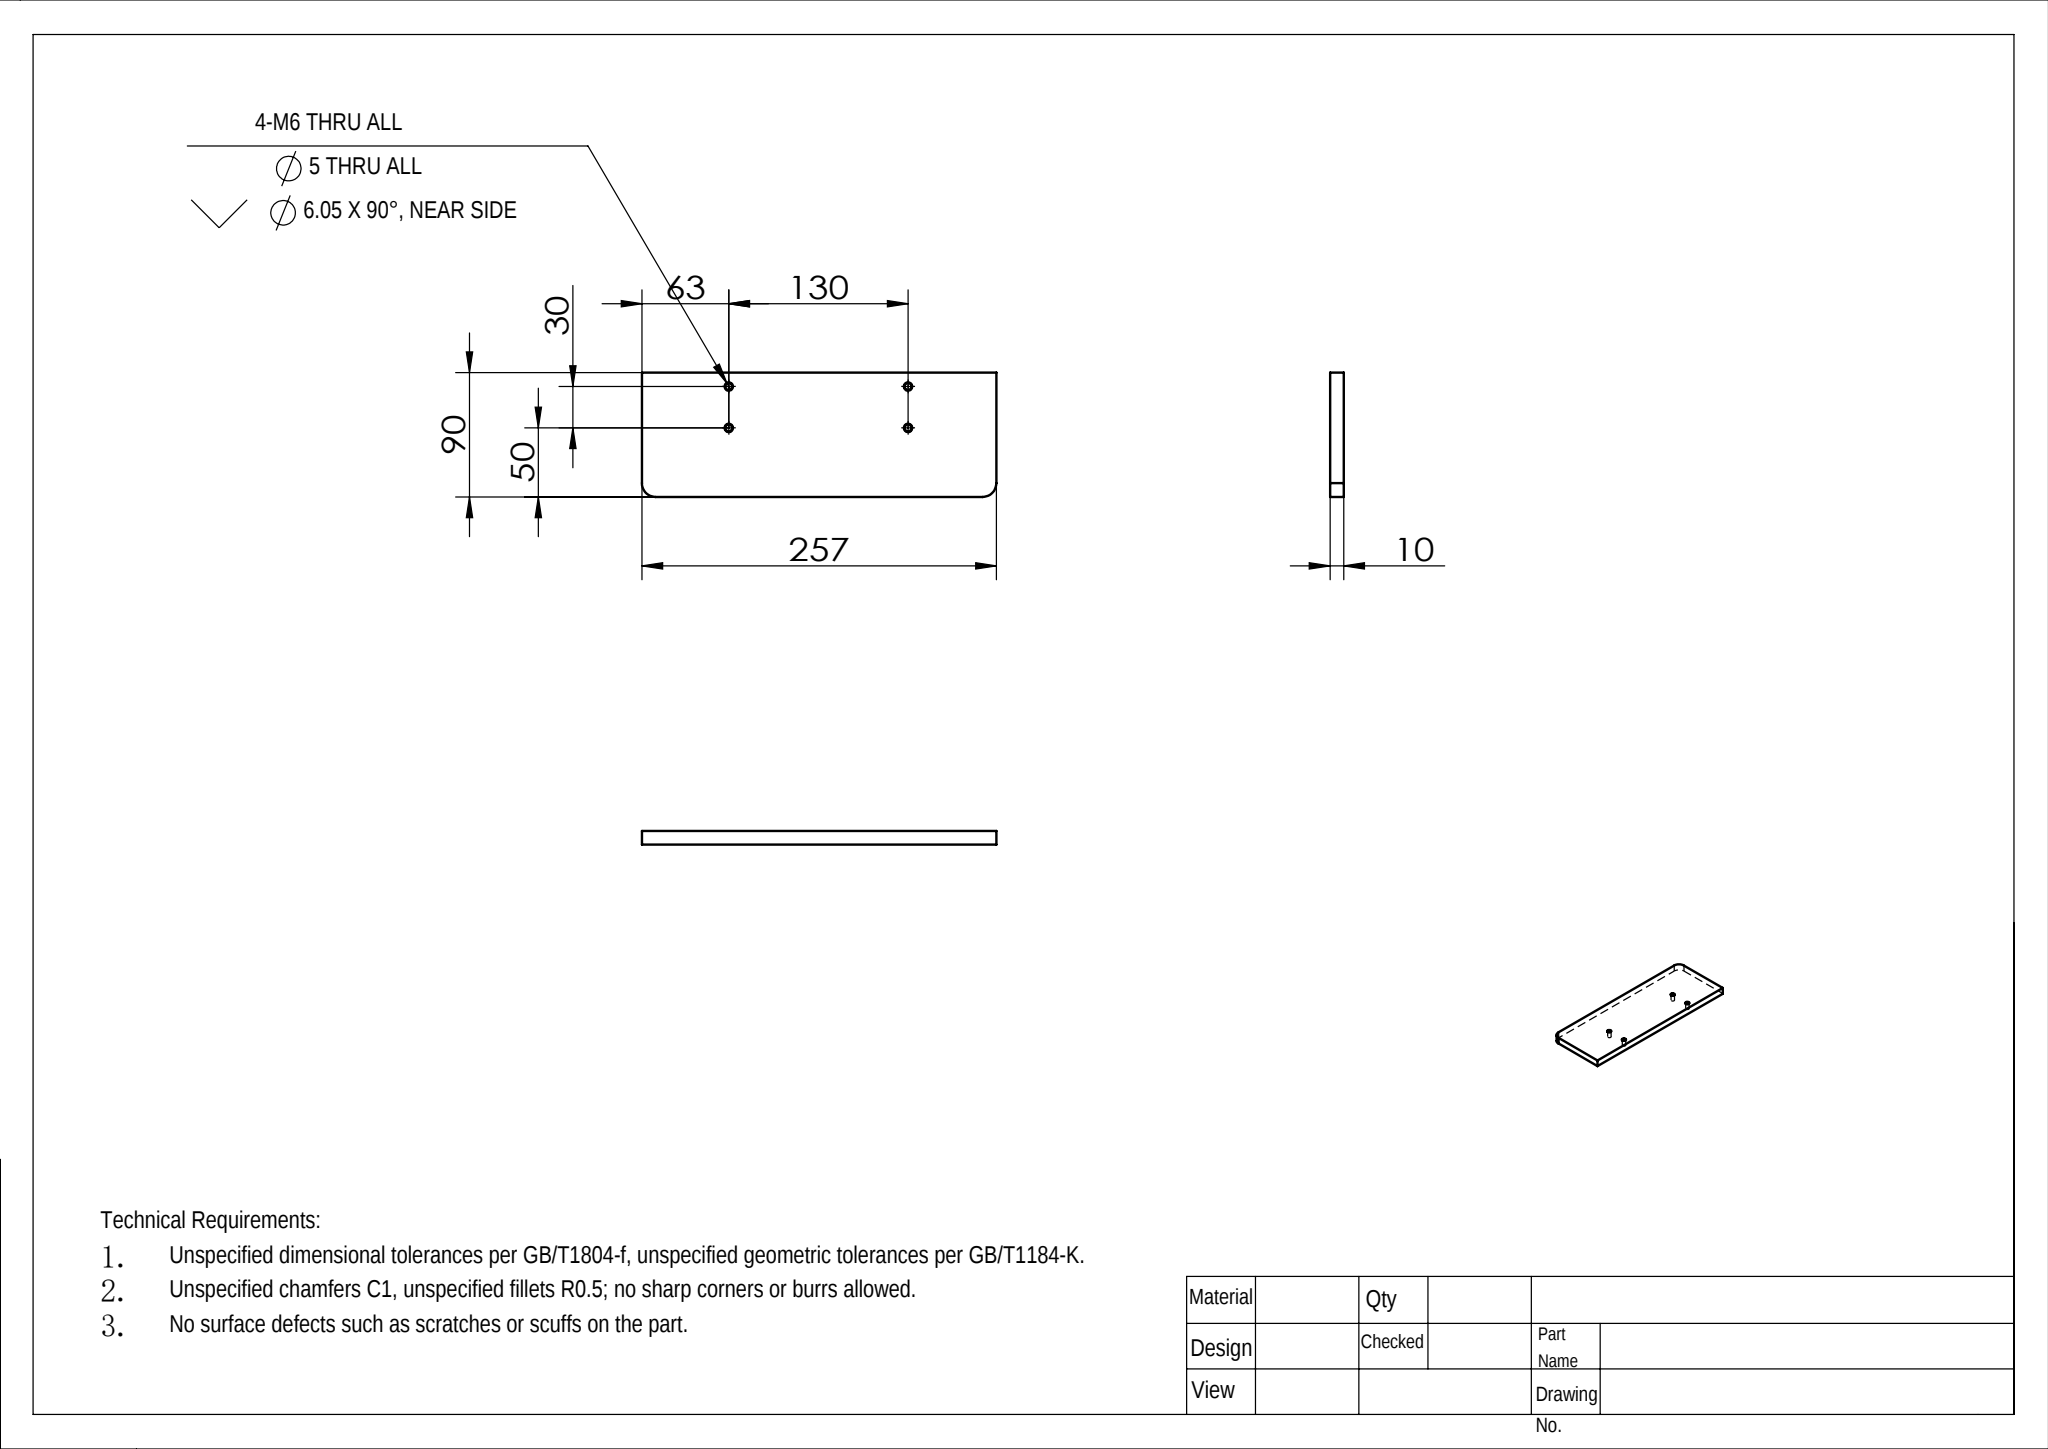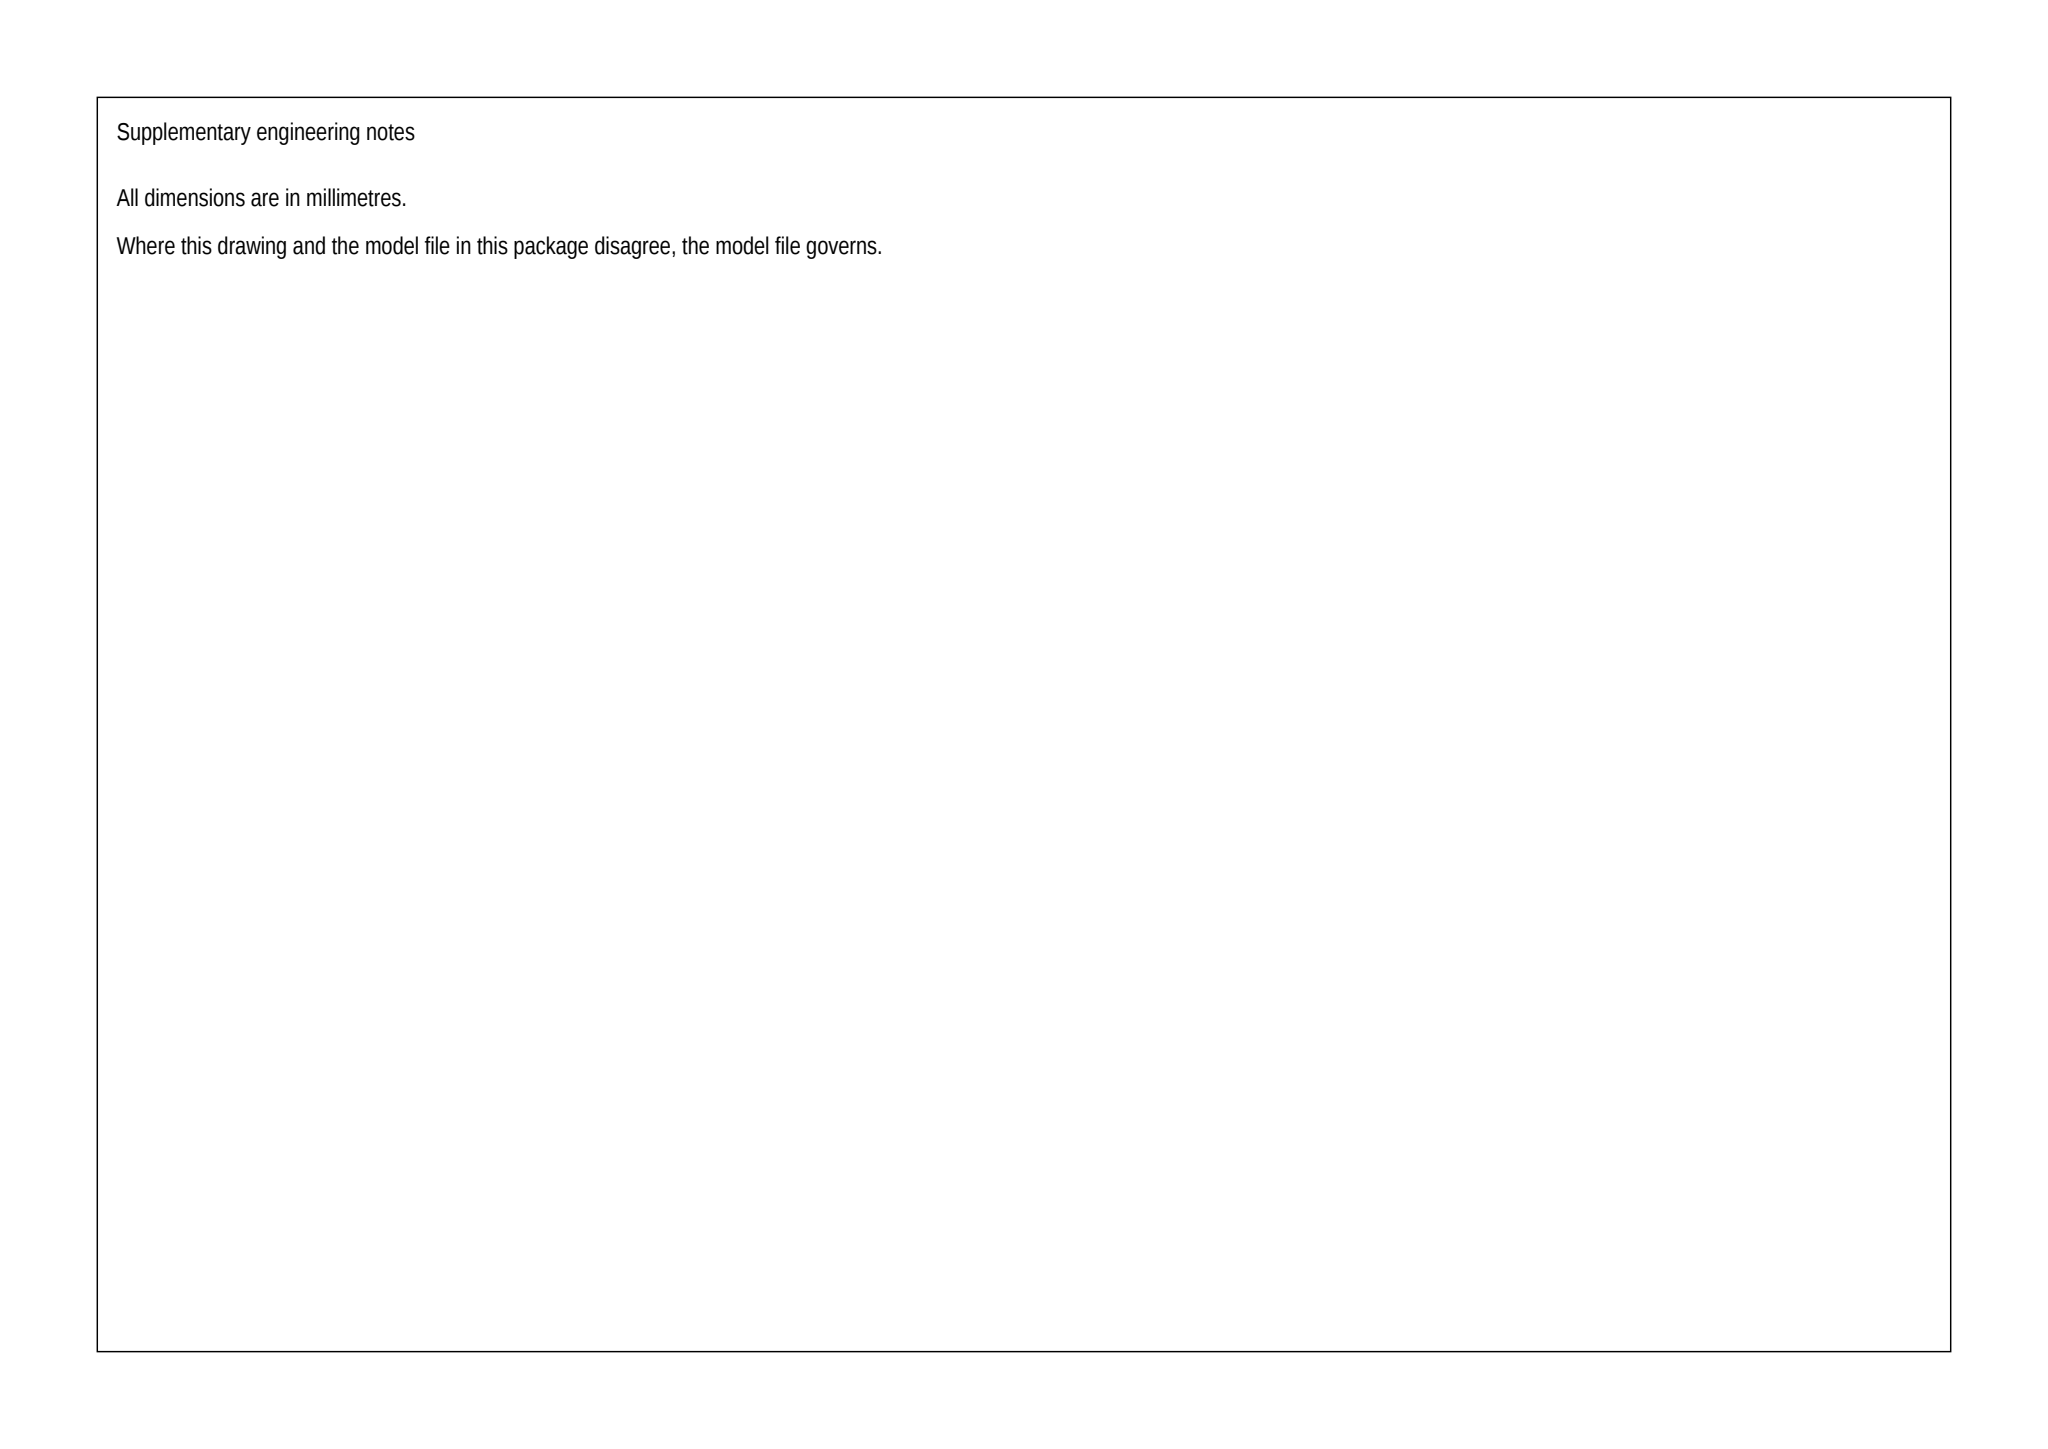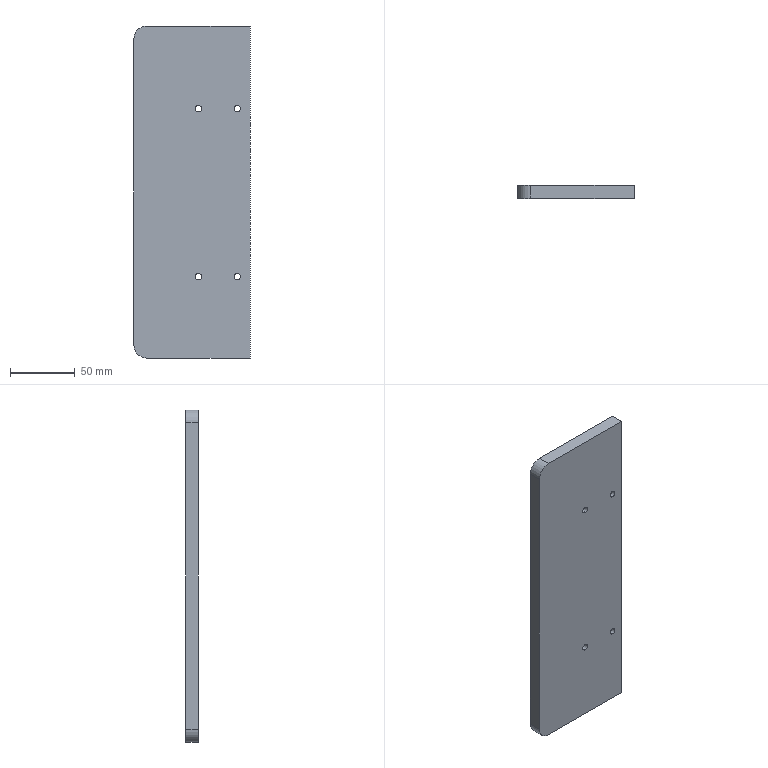Part | SolidWorks | mm | 1 solid | 24 faces | box 90 x 10 x 257 mm | volume 230076 mm3 | cylinder 10 | cone 8 | plane 6 | commonest cylinder face diameters 5 x8 20 x2
build123d program:
from build123d import *

# Parameters (mm, degrees)
SKETCH1_W                   = 90
SKETCH1_H                   = 257
BOSS_EXTRUDE1_DEPTH         = 10
FILLET1_R                   = 10
M6_TAPPED_HOLE1_D           = 5
M6_TAPPED_HOLE1_CSINK_D     = 6.05
M6_TAPPED_HOLE1_CSINK_ANGLE = 90


with BuildPart() as part:
    # Sketch1 → Boss-Extrude1 (new body)
    with BuildSketch(Plane(origin=(0, 0, 0), x_dir=(1, 0, 0), z_dir=(0, 1, 0))):
        with Locations((45, 128.5)):
            Rectangle(SKETCH1_W, SKETCH1_H)
    extrude(amount=BOSS_EXTRUDE1_DEPTH)

    # Fillet1
    fillet1_edges = [part.edges().sort_by_distance(p)[0] for p in [
        (0, 5, -257),
        (0, 5, 0),
    ]]
    fillet(fillet1_edges, radius=FILLET1_R)

    # M6 Tapped Hole1 (through all)
    with Locations(Plane(origin=(0, 10, 0), x_dir=(1, 0, 0), z_dir=(0, 1, 0))):
        with Locations((50, 64), (80, 64), (50, 194), (80, 194)):
            CounterSinkHole(M6_TAPPED_HOLE1_D / 2, M6_TAPPED_HOLE1_CSINK_D / 2, counter_sink_angle=M6_TAPPED_HOLE1_CSINK_ANGLE)


solid = part.part
STEP:
#1=CARTESIAN_POINT('',(50.,9.475,-66.5));
#2=VERTEX_POINT('',#1);
#3=CARTESIAN_POINT('',(50.,9.475,-61.5));
#4=VERTEX_POINT('',#3);
#5=CARTESIAN_POINT('',(50.,9.475,-64.));
#6=DIRECTION('',(0.,1.,0.));
#7=DIRECTION('',(0.,0.,1.));
#8=AXIS2_PLACEMENT_3D('',#5,#6,#7);
#9=CIRCLE('',#8,2.5);
#10=EDGE_CURVE('',#2,#4,#9,.T.);
#11=ORIENTED_EDGE('',*,*,#10,.F.);
#12=CARTESIAN_POINT('',(50.,10.,-67.025));
#13=VERTEX_POINT('',#12);
#14=CARTESIAN_POINT('',(50.,10.,-67.025));
#15=DIRECTION('',(0.,0.7071,-0.7071));
#16=VECTOR('',#15,1000.);
#17=LINE('',#14,#16);
#18=EDGE_CURVE('',#2,#13,#17,.T.);
#19=ORIENTED_EDGE('',*,*,#18,.T.);
#20=CARTESIAN_POINT('',(50.,10.,-60.975));
#21=VERTEX_POINT('',#20);
#22=CARTESIAN_POINT('',(50.,10.,-64.));
#23=DIRECTION('',(0.,1.,0.));
#24=DIRECTION('',(0.,0.,1.));
#25=AXIS2_PLACEMENT_3D('',#22,#23,#24);
#26=CIRCLE('',#25,3.025);
#27=EDGE_CURVE('',#13,#21,#26,.T.);
#28=ORIENTED_EDGE('',*,*,#27,.T.);
#29=CARTESIAN_POINT('',(50.,10.,-60.975));
#30=DIRECTION('',(0.,0.7071,0.7071));
#31=VECTOR('',#30,1000.);
#32=LINE('',#29,#31);
#33=EDGE_CURVE('',#4,#21,#32,.T.);
#34=ORIENTED_EDGE('',*,*,#33,.F.);
#35=EDGE_LOOP('',(#11,#19,#28,#34));
#36=FACE_OUTER_BOUND('',#35,.T.);
#37=CARTESIAN_POINT('',(50.,10.,-64.));
#38=DIRECTION('',(0.,1.,0.));
#39=DIRECTION('',(0.,0.,1.));
#40=AXIS2_PLACEMENT_3D('',#37,#38,#39);
#41=CONICAL_SURFACE('',#40,3.025,0.7854);
#42=ADVANCED_FACE('',(#36),#41,.F.);
#43=CARTESIAN_POINT('',(50.,0.,-66.5));
#44=VERTEX_POINT('',#43);
#45=CARTESIAN_POINT('',(50.,0.,-61.5));
#46=VERTEX_POINT('',#45);
#47=CARTESIAN_POINT('',(50.,0.,-64.));
#48=DIRECTION('',(0.,1.,0.));
#49=DIRECTION('',(0.,0.,1.));
#50=AXIS2_PLACEMENT_3D('',#47,#48,#49);
#51=CIRCLE('',#50,2.5);
#52=EDGE_CURVE('',#44,#46,#51,.T.);
#53=ORIENTED_EDGE('',*,*,#52,.F.);
#54=CARTESIAN_POINT('',(50.,10.,-66.5));
#55=DIRECTION('',(0.,1.,0.));
#56=VECTOR('',#55,1000.);
#57=LINE('',#54,#56);
#58=EDGE_CURVE('',#44,#2,#57,.T.);
#59=ORIENTED_EDGE('',*,*,#58,.T.);
#60=ORIENTED_EDGE('',*,*,#10,.T.);
#61=CARTESIAN_POINT('',(50.,10.,-61.5));
#62=DIRECTION('',(0.,1.,0.));
#63=VECTOR('',#62,1000.);
#64=LINE('',#61,#63);
#65=EDGE_CURVE('',#46,#4,#64,.T.);
#66=ORIENTED_EDGE('',*,*,#65,.F.);
#67=EDGE_LOOP('',(#53,#59,#60,#66));
#68=FACE_OUTER_BOUND('',#67,.T.);
#69=CARTESIAN_POINT('',(50.,10.,-64.));
#70=DIRECTION('',(0.,1.,0.));
#71=DIRECTION('',(0.,0.,1.));
#72=AXIS2_PLACEMENT_3D('',#69,#70,#71);
#73=CYLINDRICAL_SURFACE('',#72,2.5);
#74=ADVANCED_FACE('',(#68),#73,.F.);
#75=CARTESIAN_POINT('',(80.,9.475,-66.5));
#76=VERTEX_POINT('',#75);
#77=CARTESIAN_POINT('',(80.,9.475,-61.5));
#78=VERTEX_POINT('',#77);
#79=CARTESIAN_POINT('',(80.,9.475,-64.));
#80=DIRECTION('',(0.,1.,0.));
#81=DIRECTION('',(0.,0.,1.));
#82=AXIS2_PLACEMENT_3D('',#79,#80,#81);
#83=CIRCLE('',#82,2.5);
#84=EDGE_CURVE('',#76,#78,#83,.T.);
#85=ORIENTED_EDGE('',*,*,#84,.F.);
#86=CARTESIAN_POINT('',(80.,10.,-67.025));
#87=VERTEX_POINT('',#86);
#88=CARTESIAN_POINT('',(80.,10.,-67.025));
#89=DIRECTION('',(0.,0.7071,-0.7071));
#90=VECTOR('',#89,1000.);
#91=LINE('',#88,#90);
#92=EDGE_CURVE('',#76,#87,#91,.T.);
#93=ORIENTED_EDGE('',*,*,#92,.T.);
#94=CARTESIAN_POINT('',(80.,10.,-60.975));
#95=VERTEX_POINT('',#94);
#96=CARTESIAN_POINT('',(80.,10.,-64.));
#97=DIRECTION('',(0.,1.,0.));
#98=DIRECTION('',(0.,0.,1.));
#99=AXIS2_PLACEMENT_3D('',#96,#97,#98);
#100=CIRCLE('',#99,3.025);
#101=EDGE_CURVE('',#87,#95,#100,.T.);
#102=ORIENTED_EDGE('',*,*,#101,.T.);
#103=CARTESIAN_POINT('',(80.,10.,-60.975));
#104=DIRECTION('',(0.,0.7071,0.7071));
#105=VECTOR('',#104,1000.);
#106=LINE('',#103,#105);
#107=EDGE_CURVE('',#78,#95,#106,.T.);
#108=ORIENTED_EDGE('',*,*,#107,.F.);
#109=EDGE_LOOP('',(#85,#93,#102,#108));
#110=FACE_OUTER_BOUND('',#109,.T.);
#111=CARTESIAN_POINT('',(80.,10.,-64.));
#112=DIRECTION('',(0.,1.,0.));
#113=DIRECTION('',(0.,0.,1.));
#114=AXIS2_PLACEMENT_3D('',#111,#112,#113);
#115=CONICAL_SURFACE('',#114,3.025,0.7854);
#116=ADVANCED_FACE('',(#110),#115,.F.);
#117=CARTESIAN_POINT('',(80.,0.,-66.5));
#118=VERTEX_POINT('',#117);
#119=CARTESIAN_POINT('',(80.,0.,-61.5));
#120=VERTEX_POINT('',#119);
#121=CARTESIAN_POINT('',(80.,0.,-64.));
#122=DIRECTION('',(0.,1.,0.));
#123=DIRECTION('',(0.,0.,1.));
#124=AXIS2_PLACEMENT_3D('',#121,#122,#123);
#125=CIRCLE('',#124,2.5);
#126=EDGE_CURVE('',#118,#120,#125,.T.);
#127=ORIENTED_EDGE('',*,*,#126,.F.);
#128=CARTESIAN_POINT('',(80.,10.,-66.5));
#129=DIRECTION('',(0.,1.,0.));
#130=VECTOR('',#129,1000.);
#131=LINE('',#128,#130);
#132=EDGE_CURVE('',#118,#76,#131,.T.);
#133=ORIENTED_EDGE('',*,*,#132,.T.);
#134=ORIENTED_EDGE('',*,*,#84,.T.);
#135=CARTESIAN_POINT('',(80.,10.,-61.5));
#136=DIRECTION('',(0.,1.,0.));
#137=VECTOR('',#136,1000.);
#138=LINE('',#135,#137);
#139=EDGE_CURVE('',#120,#78,#138,.T.);
#140=ORIENTED_EDGE('',*,*,#139,.F.);
#141=EDGE_LOOP('',(#127,#133,#134,#140));
#142=FACE_OUTER_BOUND('',#141,.T.);
#143=CARTESIAN_POINT('',(80.,10.,-64.));
#144=DIRECTION('',(0.,1.,0.));
#145=DIRECTION('',(0.,0.,1.));
#146=AXIS2_PLACEMENT_3D('',#143,#144,#145);
#147=CYLINDRICAL_SURFACE('',#146,2.5);
#148=ADVANCED_FACE('',(#142),#147,.F.);
#149=CARTESIAN_POINT('',(50.,9.475,-196.5));
#150=VERTEX_POINT('',#149);
#151=CARTESIAN_POINT('',(50.,9.475,-191.5));
#152=VERTEX_POINT('',#151);
#153=CARTESIAN_POINT('',(50.,9.475,-194.));
#154=DIRECTION('',(0.,1.,0.));
#155=DIRECTION('',(0.,0.,1.));
#156=AXIS2_PLACEMENT_3D('',#153,#154,#155);
#157=CIRCLE('',#156,2.5);
#158=EDGE_CURVE('',#150,#152,#157,.T.);
#159=ORIENTED_EDGE('',*,*,#158,.F.);
#160=CARTESIAN_POINT('',(50.,10.,-197.025));
#161=VERTEX_POINT('',#160);
#162=CARTESIAN_POINT('',(50.,10.,-197.025));
#163=DIRECTION('',(0.,0.7071,-0.7071));
#164=VECTOR('',#163,1000.);
#165=LINE('',#162,#164);
#166=EDGE_CURVE('',#150,#161,#165,.T.);
#167=ORIENTED_EDGE('',*,*,#166,.T.);
#168=CARTESIAN_POINT('',(50.,10.,-190.975));
#169=VERTEX_POINT('',#168);
#170=CARTESIAN_POINT('',(50.,10.,-194.));
#171=DIRECTION('',(0.,1.,0.));
#172=DIRECTION('',(0.,0.,1.));
#173=AXIS2_PLACEMENT_3D('',#170,#171,#172);
#174=CIRCLE('',#173,3.025);
#175=EDGE_CURVE('',#161,#169,#174,.T.);
#176=ORIENTED_EDGE('',*,*,#175,.T.);
#177=CARTESIAN_POINT('',(50.,10.,-190.975));
#178=DIRECTION('',(0.,0.7071,0.7071));
#179=VECTOR('',#178,1000.);
#180=LINE('',#177,#179);
#181=EDGE_CURVE('',#152,#169,#180,.T.);
#182=ORIENTED_EDGE('',*,*,#181,.F.);
#183=EDGE_LOOP('',(#159,#167,#176,#182));
#184=FACE_OUTER_BOUND('',#183,.T.);
#185=CARTESIAN_POINT('',(50.,10.,-194.));
#186=DIRECTION('',(0.,1.,0.));
#187=DIRECTION('',(0.,0.,1.));
#188=AXIS2_PLACEMENT_3D('',#185,#186,#187);
#189=CONICAL_SURFACE('',#188,3.025,0.7854);
#190=ADVANCED_FACE('',(#184),#189,.F.);
#191=CARTESIAN_POINT('',(50.,0.,-196.5));
#192=VERTEX_POINT('',#191);
#193=CARTESIAN_POINT('',(50.,0.,-191.5));
#194=VERTEX_POINT('',#193);
#195=CARTESIAN_POINT('',(50.,0.,-194.));
#196=DIRECTION('',(0.,1.,0.));
#197=DIRECTION('',(0.,0.,1.));
#198=AXIS2_PLACEMENT_3D('',#195,#196,#197);
#199=CIRCLE('',#198,2.5);
#200=EDGE_CURVE('',#192,#194,#199,.T.);
#201=ORIENTED_EDGE('',*,*,#200,.F.);
#202=CARTESIAN_POINT('',(50.,10.,-196.5));
#203=DIRECTION('',(0.,1.,0.));
#204=VECTOR('',#203,1000.);
#205=LINE('',#202,#204);
#206=EDGE_CURVE('',#192,#150,#205,.T.);
#207=ORIENTED_EDGE('',*,*,#206,.T.);
#208=ORIENTED_EDGE('',*,*,#158,.T.);
#209=CARTESIAN_POINT('',(50.,10.,-191.5));
#210=DIRECTION('',(0.,1.,0.));
#211=VECTOR('',#210,1000.);
#212=LINE('',#209,#211);
#213=EDGE_CURVE('',#194,#152,#212,.T.);
#214=ORIENTED_EDGE('',*,*,#213,.F.);
#215=EDGE_LOOP('',(#201,#207,#208,#214));
#216=FACE_OUTER_BOUND('',#215,.T.);
#217=CARTESIAN_POINT('',(50.,10.,-194.));
#218=DIRECTION('',(0.,1.,0.));
#219=DIRECTION('',(0.,0.,1.));
#220=AXIS2_PLACEMENT_3D('',#217,#218,#219);
#221=CYLINDRICAL_SURFACE('',#220,2.5);
#222=ADVANCED_FACE('',(#216),#221,.F.);
#223=CARTESIAN_POINT('',(80.,9.475,-196.5));
#224=VERTEX_POINT('',#223);
#225=CARTESIAN_POINT('',(80.,9.475,-191.5));
#226=VERTEX_POINT('',#225);
#227=CARTESIAN_POINT('',(80.,9.475,-194.));
#228=DIRECTION('',(0.,1.,0.));
#229=DIRECTION('',(0.,0.,1.));
#230=AXIS2_PLACEMENT_3D('',#227,#228,#229);
#231=CIRCLE('',#230,2.5);
#232=EDGE_CURVE('',#224,#226,#231,.T.);
#233=ORIENTED_EDGE('',*,*,#232,.F.);
#234=CARTESIAN_POINT('',(80.,10.,-197.025));
#235=VERTEX_POINT('',#234);
#236=CARTESIAN_POINT('',(80.,10.,-197.025));
#237=DIRECTION('',(0.,0.7071,-0.7071));
#238=VECTOR('',#237,1000.);
#239=LINE('',#236,#238);
#240=EDGE_CURVE('',#224,#235,#239,.T.);
#241=ORIENTED_EDGE('',*,*,#240,.T.);
#242=CARTESIAN_POINT('',(80.,10.,-190.975));
#243=VERTEX_POINT('',#242);
#244=CARTESIAN_POINT('',(80.,10.,-194.));
#245=DIRECTION('',(0.,1.,0.));
#246=DIRECTION('',(0.,0.,1.));
#247=AXIS2_PLACEMENT_3D('',#244,#245,#246);
#248=CIRCLE('',#247,3.025);
#249=EDGE_CURVE('',#235,#243,#248,.T.);
#250=ORIENTED_EDGE('',*,*,#249,.T.);
#251=CARTESIAN_POINT('',(80.,10.,-190.975));
#252=DIRECTION('',(0.,0.7071,0.7071));
#253=VECTOR('',#252,1000.);
#254=LINE('',#251,#253);
#255=EDGE_CURVE('',#226,#243,#254,.T.);
#256=ORIENTED_EDGE('',*,*,#255,.F.);
#257=EDGE_LOOP('',(#233,#241,#250,#256));
#258=FACE_OUTER_BOUND('',#257,.T.);
#259=CARTESIAN_POINT('',(80.,10.,-194.));
#260=DIRECTION('',(0.,1.,0.));
#261=DIRECTION('',(0.,0.,1.));
#262=AXIS2_PLACEMENT_3D('',#259,#260,#261);
#263=CONICAL_SURFACE('',#262,3.025,0.7854);
#264=ADVANCED_FACE('',(#258),#263,.F.);
#265=CARTESIAN_POINT('',(80.,0.,-196.5));
#266=VERTEX_POINT('',#265);
#267=CARTESIAN_POINT('',(80.,0.,-191.5));
#268=VERTEX_POINT('',#267);
#269=CARTESIAN_POINT('',(80.,0.,-194.));
#270=DIRECTION('',(0.,1.,0.));
#271=DIRECTION('',(0.,0.,1.));
#272=AXIS2_PLACEMENT_3D('',#269,#270,#271);
#273=CIRCLE('',#272,2.5);
#274=EDGE_CURVE('',#266,#268,#273,.T.);
#275=ORIENTED_EDGE('',*,*,#274,.F.);
#276=CARTESIAN_POINT('',(80.,10.,-196.5));
#277=DIRECTION('',(0.,1.,0.));
#278=VECTOR('',#277,1000.);
#279=LINE('',#276,#278);
#280=EDGE_CURVE('',#266,#224,#279,.T.);
#281=ORIENTED_EDGE('',*,*,#280,.T.);
#282=ORIENTED_EDGE('',*,*,#232,.T.);
#283=CARTESIAN_POINT('',(80.,10.,-191.5));
#284=DIRECTION('',(0.,1.,0.));
#285=VECTOR('',#284,1000.);
#286=LINE('',#283,#285);
#287=EDGE_CURVE('',#268,#226,#286,.T.);
#288=ORIENTED_EDGE('',*,*,#287,.F.);
#289=EDGE_LOOP('',(#275,#281,#282,#288));
#290=FACE_OUTER_BOUND('',#289,.T.);
#291=CARTESIAN_POINT('',(80.,10.,-194.));
#292=DIRECTION('',(0.,1.,0.));
#293=DIRECTION('',(0.,0.,1.));
#294=AXIS2_PLACEMENT_3D('',#291,#292,#293);
#295=CYLINDRICAL_SURFACE('',#294,2.5);
#296=ADVANCED_FACE('',(#290),#295,.F.);
#297=CARTESIAN_POINT('',(0.,0.,-247.));
#298=VERTEX_POINT('',#297);
#299=CARTESIAN_POINT('',(0.,0.,-10.));
#300=VERTEX_POINT('',#299);
#301=CARTESIAN_POINT('',(0.,0.,0.));
#302=DIRECTION('',(0.,0.,1.));
#303=VECTOR('',#302,1000.);
#304=LINE('',#301,#303);
#305=EDGE_CURVE('',#298,#300,#304,.T.);
#306=ORIENTED_EDGE('',*,*,#305,.T.);
#307=CARTESIAN_POINT('',(0.,10.,-10.));
#308=VERTEX_POINT('',#307);
#309=CARTESIAN_POINT('',(0.,10.,-10.));
#310=DIRECTION('',(0.,1.,0.));
#311=VECTOR('',#310,1000.);
#312=LINE('',#309,#311);
#313=EDGE_CURVE('',#300,#308,#312,.T.);
#314=ORIENTED_EDGE('',*,*,#313,.T.);
#315=CARTESIAN_POINT('',(0.,10.,-247.));
#316=VERTEX_POINT('',#315);
#317=CARTESIAN_POINT('',(0.,10.,0.));
#318=DIRECTION('',(0.,0.,1.));
#319=VECTOR('',#318,1000.);
#320=LINE('',#317,#319);
#321=EDGE_CURVE('',#316,#308,#320,.T.);
#322=ORIENTED_EDGE('',*,*,#321,.F.);
#323=CARTESIAN_POINT('',(0.,10.,-247.));
#324=DIRECTION('',(0.,-1.,0.));
#325=VECTOR('',#324,1000.);
#326=LINE('',#323,#325);
#327=EDGE_CURVE('',#316,#298,#326,.T.);
#328=ORIENTED_EDGE('',*,*,#327,.T.);
#329=EDGE_LOOP('',(#306,#314,#322,#328));
#330=FACE_OUTER_BOUND('',#329,.T.);
#331=CARTESIAN_POINT('',(0.,10.,0.));
#332=DIRECTION('',(1.,0.,0.));
#333=DIRECTION('',(0.,0.,-1.));
#334=AXIS2_PLACEMENT_3D('',#331,#332,#333);
#335=PLANE('',#334);
#336=ADVANCED_FACE('',(#330),#335,.F.);
#337=CARTESIAN_POINT('',(10.,10.,0.));
#338=VERTEX_POINT('',#337);
#339=CARTESIAN_POINT('',(90.,10.,0.));
#340=VERTEX_POINT('',#339);
#341=CARTESIAN_POINT('',(0.,10.,0.));
#342=DIRECTION('',(1.,0.,0.));
#343=VECTOR('',#342,1000.);
#344=LINE('',#341,#343);
#345=EDGE_CURVE('',#338,#340,#344,.T.);
#346=ORIENTED_EDGE('',*,*,#345,.F.);
#347=CARTESIAN_POINT('',(10.,0.,0.));
#348=VERTEX_POINT('',#347);
#349=CARTESIAN_POINT('',(10.,10.,0.));
#350=DIRECTION('',(0.,-1.,0.));
#351=VECTOR('',#350,1000.);
#352=LINE('',#349,#351);
#353=EDGE_CURVE('',#338,#348,#352,.T.);
#354=ORIENTED_EDGE('',*,*,#353,.T.);
#355=CARTESIAN_POINT('',(90.,0.,0.));
#356=VERTEX_POINT('',#355);
#357=CARTESIAN_POINT('',(0.,0.,0.));
#358=DIRECTION('',(1.,0.,0.));
#359=VECTOR('',#358,1000.);
#360=LINE('',#357,#359);
#361=EDGE_CURVE('',#348,#356,#360,.T.);
#362=ORIENTED_EDGE('',*,*,#361,.T.);
#363=CARTESIAN_POINT('',(90.,10.,0.));
#364=DIRECTION('',(0.,-1.,0.));
#365=VECTOR('',#364,1000.);
#366=LINE('',#363,#365);
#367=EDGE_CURVE('',#340,#356,#366,.T.);
#368=ORIENTED_EDGE('',*,*,#367,.F.);
#369=EDGE_LOOP('',(#346,#354,#362,#368));
#370=FACE_OUTER_BOUND('',#369,.T.);
#371=CARTESIAN_POINT('',(0.,10.,0.));
#372=DIRECTION('',(0.,0.,-1.));
#373=DIRECTION('',(-1.,0.,0.));
#374=AXIS2_PLACEMENT_3D('',#371,#372,#373);
#375=PLANE('',#374);
#376=ADVANCED_FACE('',(#370),#375,.F.);
#377=CARTESIAN_POINT('',(90.,0.,-257.));
#378=VERTEX_POINT('',#377);
#379=CARTESIAN_POINT('',(90.,0.,0.));
#380=DIRECTION('',(0.,0.,-1.));
#381=VECTOR('',#380,1000.);
#382=LINE('',#379,#381);
#383=EDGE_CURVE('',#356,#378,#382,.T.);
#384=ORIENTED_EDGE('',*,*,#383,.T.);
#385=CARTESIAN_POINT('',(90.,10.,-257.));
#386=VERTEX_POINT('',#385);
#387=CARTESIAN_POINT('',(90.,10.,-257.));
#388=DIRECTION('',(0.,-1.,0.));
#389=VECTOR('',#388,1000.);
#390=LINE('',#387,#389);
#391=EDGE_CURVE('',#386,#378,#390,.T.);
#392=ORIENTED_EDGE('',*,*,#391,.F.);
#393=CARTESIAN_POINT('',(90.,10.,0.));
#394=DIRECTION('',(0.,0.,-1.));
#395=VECTOR('',#394,1000.);
#396=LINE('',#393,#395);
#397=EDGE_CURVE('',#340,#386,#396,.T.);
#398=ORIENTED_EDGE('',*,*,#397,.F.);
#399=ORIENTED_EDGE('',*,*,#367,.T.);
#400=EDGE_LOOP('',(#384,#392,#398,#399));
#401=FACE_OUTER_BOUND('',#400,.T.);
#402=CARTESIAN_POINT('',(90.,10.,0.));
#403=DIRECTION('',(-1.,0.,0.));
#404=DIRECTION('',(0.,0.,1.));
#405=AXIS2_PLACEMENT_3D('',#402,#403,#404);
#406=PLANE('',#405);
#407=ADVANCED_FACE('',(#401),#406,.F.);
#408=CARTESIAN_POINT('',(10.,0.,-257.));
#409=VERTEX_POINT('',#408);
#410=CARTESIAN_POINT('',(0.,0.,-257.));
#411=DIRECTION('',(-1.,0.,0.));
#412=VECTOR('',#411,1000.);
#413=LINE('',#410,#412);
#414=EDGE_CURVE('',#378,#409,#413,.T.);
#415=ORIENTED_EDGE('',*,*,#414,.T.);
#416=CARTESIAN_POINT('',(10.,10.,-257.));
#417=VERTEX_POINT('',#416);
#418=CARTESIAN_POINT('',(10.,10.,-257.));
#419=DIRECTION('',(0.,1.,0.));
#420=VECTOR('',#419,1000.);
#421=LINE('',#418,#420);
#422=EDGE_CURVE('',#409,#417,#421,.T.);
#423=ORIENTED_EDGE('',*,*,#422,.T.);
#424=CARTESIAN_POINT('',(0.,10.,-257.));
#425=DIRECTION('',(-1.,0.,0.));
#426=VECTOR('',#425,1000.);
#427=LINE('',#424,#426);
#428=EDGE_CURVE('',#386,#417,#427,.T.);
#429=ORIENTED_EDGE('',*,*,#428,.F.);
#430=ORIENTED_EDGE('',*,*,#391,.T.);
#431=EDGE_LOOP('',(#415,#423,#429,#430));
#432=FACE_OUTER_BOUND('',#431,.T.);
#433=CARTESIAN_POINT('',(0.,10.,-257.));
#434=DIRECTION('',(0.,0.,1.));
#435=DIRECTION('',(1.,0.,0.));
#436=AXIS2_PLACEMENT_3D('',#433,#434,#435);
#437=PLANE('',#436);
#438=ADVANCED_FACE('',(#432),#437,.F.);
#439=CARTESIAN_POINT('',(50.,10.,-64.));
#440=DIRECTION('',(0.,1.,0.));
#441=DIRECTION('',(0.,0.,1.));
#442=AXIS2_PLACEMENT_3D('',#439,#440,#441);
#443=CIRCLE('',#442,3.025);
#444=EDGE_CURVE('',#21,#13,#443,.T.);
#445=ORIENTED_EDGE('',*,*,#444,.F.);
#446=ORIENTED_EDGE('',*,*,#27,.F.);
#447=EDGE_LOOP('',(#445,#446));
#448=FACE_BOUND('',#447,.T.);
#449=CARTESIAN_POINT('',(80.,10.,-64.));
#450=DIRECTION('',(0.,1.,0.));
#451=DIRECTION('',(0.,0.,1.));
#452=AXIS2_PLACEMENT_3D('',#449,#450,#451);
#453=CIRCLE('',#452,3.025);
#454=EDGE_CURVE('',#95,#87,#453,.T.);
#455=ORIENTED_EDGE('',*,*,#454,.F.);
#456=ORIENTED_EDGE('',*,*,#101,.F.);
#457=EDGE_LOOP('',(#455,#456));
#458=FACE_BOUND('',#457,.T.);
#459=CARTESIAN_POINT('',(50.,10.,-194.));
#460=DIRECTION('',(0.,1.,0.));
#461=DIRECTION('',(0.,0.,1.));
#462=AXIS2_PLACEMENT_3D('',#459,#460,#461);
#463=CIRCLE('',#462,3.025);
#464=EDGE_CURVE('',#169,#161,#463,.T.);
#465=ORIENTED_EDGE('',*,*,#464,.F.);
#466=ORIENTED_EDGE('',*,*,#175,.F.);
#467=EDGE_LOOP('',(#465,#466));
#468=FACE_BOUND('',#467,.T.);
#469=CARTESIAN_POINT('',(80.,10.,-194.));
#470=DIRECTION('',(0.,1.,0.));
#471=DIRECTION('',(0.,0.,1.));
#472=AXIS2_PLACEMENT_3D('',#469,#470,#471);
#473=CIRCLE('',#472,3.025);
#474=EDGE_CURVE('',#243,#235,#473,.T.);
#475=ORIENTED_EDGE('',*,*,#474,.F.);
#476=ORIENTED_EDGE('',*,*,#249,.F.);
#477=EDGE_LOOP('',(#475,#476));
#478=FACE_BOUND('',#477,.T.);
#479=ORIENTED_EDGE('',*,*,#321,.T.);
#480=CARTESIAN_POINT('',(10.,10.,-10.));
#481=DIRECTION('',(0.,1.,0.));
#482=DIRECTION('',(0.,0.,-1.));
#483=AXIS2_PLACEMENT_3D('',#480,#481,#482);
#484=CIRCLE('',#483,10.);
#485=EDGE_CURVE('',#308,#338,#484,.T.);
#486=ORIENTED_EDGE('',*,*,#485,.T.);
#487=ORIENTED_EDGE('',*,*,#345,.T.);
#488=ORIENTED_EDGE('',*,*,#397,.T.);
#489=ORIENTED_EDGE('',*,*,#428,.T.);
#490=CARTESIAN_POINT('',(10.,10.,-247.));
#491=DIRECTION('',(0.,1.,0.));
#492=DIRECTION('',(0.,0.,-1.));
#493=AXIS2_PLACEMENT_3D('',#490,#491,#492);
#494=CIRCLE('',#493,10.);
#495=EDGE_CURVE('',#417,#316,#494,.T.);
#496=ORIENTED_EDGE('',*,*,#495,.T.);
#497=EDGE_LOOP('',(#479,#486,#487,#488,#489,#496));
#498=FACE_OUTER_BOUND('',#497,.T.);
#499=CARTESIAN_POINT('',(0.,10.,0.));
#500=DIRECTION('',(0.,-1.,0.));
#501=DIRECTION('',(0.,0.,-1.));
#502=AXIS2_PLACEMENT_3D('',#499,#500,#501);
#503=PLANE('',#502);
#504=ADVANCED_FACE('',(#448,#458,#468,#478,#498),#503,.F.);
#505=CARTESIAN_POINT('',(50.,0.,-64.));
#506=DIRECTION('',(0.,1.,0.));
#507=DIRECTION('',(0.,0.,1.));
#508=AXIS2_PLACEMENT_3D('',#505,#506,#507);
#509=CIRCLE('',#508,2.5);
#510=EDGE_CURVE('',#46,#44,#509,.T.);
#511=ORIENTED_EDGE('',*,*,#510,.T.);
#512=ORIENTED_EDGE('',*,*,#52,.T.);
#513=EDGE_LOOP('',(#511,#512));
#514=FACE_BOUND('',#513,.T.);
#515=CARTESIAN_POINT('',(80.,0.,-64.));
#516=DIRECTION('',(0.,1.,0.));
#517=DIRECTION('',(0.,0.,1.));
#518=AXIS2_PLACEMENT_3D('',#515,#516,#517);
#519=CIRCLE('',#518,2.5);
#520=EDGE_CURVE('',#120,#118,#519,.T.);
#521=ORIENTED_EDGE('',*,*,#520,.T.);
#522=ORIENTED_EDGE('',*,*,#126,.T.);
#523=EDGE_LOOP('',(#521,#522));
#524=FACE_BOUND('',#523,.T.);
#525=CARTESIAN_POINT('',(50.,0.,-194.));
#526=DIRECTION('',(0.,1.,0.));
#527=DIRECTION('',(0.,0.,1.));
#528=AXIS2_PLACEMENT_3D('',#525,#526,#527);
#529=CIRCLE('',#528,2.5);
#530=EDGE_CURVE('',#194,#192,#529,.T.);
#531=ORIENTED_EDGE('',*,*,#530,.T.);
#532=ORIENTED_EDGE('',*,*,#200,.T.);
#533=EDGE_LOOP('',(#531,#532));
#534=FACE_BOUND('',#533,.T.);
#535=CARTESIAN_POINT('',(80.,0.,-194.));
#536=DIRECTION('',(0.,1.,0.));
#537=DIRECTION('',(0.,0.,1.));
#538=AXIS2_PLACEMENT_3D('',#535,#536,#537);
#539=CIRCLE('',#538,2.5);
#540=EDGE_CURVE('',#268,#266,#539,.T.);
#541=ORIENTED_EDGE('',*,*,#540,.T.);
#542=ORIENTED_EDGE('',*,*,#274,.T.);
#543=EDGE_LOOP('',(#541,#542));
#544=FACE_BOUND('',#543,.T.);
#545=ORIENTED_EDGE('',*,*,#361,.F.);
#546=CARTESIAN_POINT('',(10.,0.,-10.));
#547=DIRECTION('',(0.,-1.,0.));
#548=DIRECTION('',(0.,0.,-1.));
#549=AXIS2_PLACEMENT_3D('',#546,#547,#548);
#550=CIRCLE('',#549,10.);
#551=EDGE_CURVE('',#348,#300,#550,.T.);
#552=ORIENTED_EDGE('',*,*,#551,.T.);
#553=ORIENTED_EDGE('',*,*,#305,.F.);
#554=CARTESIAN_POINT('',(10.,0.,-247.));
#555=DIRECTION('',(0.,-1.,0.));
#556=DIRECTION('',(0.,0.,-1.));
#557=AXIS2_PLACEMENT_3D('',#554,#555,#556);
#558=CIRCLE('',#557,10.);
#559=EDGE_CURVE('',#298,#409,#558,.T.);
#560=ORIENTED_EDGE('',*,*,#559,.T.);
#561=ORIENTED_EDGE('',*,*,#414,.F.);
#562=ORIENTED_EDGE('',*,*,#383,.F.);
#563=EDGE_LOOP('',(#545,#552,#553,#560,#561,#562));
#564=FACE_OUTER_BOUND('',#563,.T.);
#565=CARTESIAN_POINT('',(0.,0.,0.));
#566=DIRECTION('',(0.,-1.,0.));
#567=DIRECTION('',(0.,0.,-1.));
#568=AXIS2_PLACEMENT_3D('',#565,#566,#567);
#569=PLANE('',#568);
#570=ADVANCED_FACE('',(#514,#524,#534,#544,#564),#569,.T.);
#571=ORIENTED_EDGE('',*,*,#485,.F.);
#572=ORIENTED_EDGE('',*,*,#313,.F.);
#573=ORIENTED_EDGE('',*,*,#551,.F.);
#574=ORIENTED_EDGE('',*,*,#353,.F.);
#575=EDGE_LOOP('',(#571,#572,#573,#574));
#576=FACE_OUTER_BOUND('',#575,.T.);
#577=CARTESIAN_POINT('',(10.,10.,-10.));
#578=DIRECTION('',(0.,-1.,0.));
#579=DIRECTION('',(0.,0.,-1.));
#580=AXIS2_PLACEMENT_3D('',#577,#578,#579);
#581=CYLINDRICAL_SURFACE('',#580,10.);
#582=ADVANCED_FACE('',(#576),#581,.T.);
#583=ORIENTED_EDGE('',*,*,#495,.F.);
#584=ORIENTED_EDGE('',*,*,#422,.F.);
#585=ORIENTED_EDGE('',*,*,#559,.F.);
#586=ORIENTED_EDGE('',*,*,#327,.F.);
#587=EDGE_LOOP('',(#583,#584,#585,#586));
#588=FACE_OUTER_BOUND('',#587,.T.);
#589=CARTESIAN_POINT('',(10.,10.,-247.));
#590=DIRECTION('',(0.,-1.,0.));
#591=DIRECTION('',(0.,0.,-1.));
#592=AXIS2_PLACEMENT_3D('',#589,#590,#591);
#593=CYLINDRICAL_SURFACE('',#592,10.);
#594=ADVANCED_FACE('',(#588),#593,.T.);
#595=ORIENTED_EDGE('',*,*,#280,.F.);
#596=ORIENTED_EDGE('',*,*,#540,.F.);
#597=ORIENTED_EDGE('',*,*,#287,.T.);
#598=CARTESIAN_POINT('',(80.,9.475,-194.));
#599=DIRECTION('',(0.,1.,0.));
#600=DIRECTION('',(0.,0.,1.));
#601=AXIS2_PLACEMENT_3D('',#598,#599,#600);
#602=CIRCLE('',#601,2.5);
#603=EDGE_CURVE('',#226,#224,#602,.T.);
#604=ORIENTED_EDGE('',*,*,#603,.T.);
#605=EDGE_LOOP('',(#595,#596,#597,#604));
#606=FACE_OUTER_BOUND('',#605,.T.);
#607=CARTESIAN_POINT('',(80.,10.,-194.));
#608=DIRECTION('',(0.,1.,0.));
#609=DIRECTION('',(0.,0.,1.));
#610=AXIS2_PLACEMENT_3D('',#607,#608,#609);
#611=CYLINDRICAL_SURFACE('',#610,2.5);
#612=ADVANCED_FACE('',(#606),#611,.F.);
#613=ORIENTED_EDGE('',*,*,#240,.F.);
#614=ORIENTED_EDGE('',*,*,#603,.F.);
#615=ORIENTED_EDGE('',*,*,#255,.T.);
#616=ORIENTED_EDGE('',*,*,#474,.T.);
#617=EDGE_LOOP('',(#613,#614,#615,#616));
#618=FACE_OUTER_BOUND('',#617,.T.);
#619=CARTESIAN_POINT('',(80.,10.,-194.));
#620=DIRECTION('',(0.,1.,0.));
#621=DIRECTION('',(0.,0.,1.));
#622=AXIS2_PLACEMENT_3D('',#619,#620,#621);
#623=CONICAL_SURFACE('',#622,3.025,0.7854);
#624=ADVANCED_FACE('',(#618),#623,.F.);
#625=ORIENTED_EDGE('',*,*,#206,.F.);
#626=ORIENTED_EDGE('',*,*,#530,.F.);
#627=ORIENTED_EDGE('',*,*,#213,.T.);
#628=CARTESIAN_POINT('',(50.,9.475,-194.));
#629=DIRECTION('',(0.,1.,0.));
#630=DIRECTION('',(0.,0.,1.));
#631=AXIS2_PLACEMENT_3D('',#628,#629,#630);
#632=CIRCLE('',#631,2.5);
#633=EDGE_CURVE('',#152,#150,#632,.T.);
#634=ORIENTED_EDGE('',*,*,#633,.T.);
#635=EDGE_LOOP('',(#625,#626,#627,#634));
#636=FACE_OUTER_BOUND('',#635,.T.);
#637=CARTESIAN_POINT('',(50.,10.,-194.));
#638=DIRECTION('',(0.,1.,0.));
#639=DIRECTION('',(0.,0.,1.));
#640=AXIS2_PLACEMENT_3D('',#637,#638,#639);
#641=CYLINDRICAL_SURFACE('',#640,2.5);
#642=ADVANCED_FACE('',(#636),#641,.F.);
#643=ORIENTED_EDGE('',*,*,#166,.F.);
#644=ORIENTED_EDGE('',*,*,#633,.F.);
#645=ORIENTED_EDGE('',*,*,#181,.T.);
#646=ORIENTED_EDGE('',*,*,#464,.T.);
#647=EDGE_LOOP('',(#643,#644,#645,#646));
#648=FACE_OUTER_BOUND('',#647,.T.);
#649=CARTESIAN_POINT('',(50.,10.,-194.));
#650=DIRECTION('',(0.,1.,0.));
#651=DIRECTION('',(0.,0.,1.));
#652=AXIS2_PLACEMENT_3D('',#649,#650,#651);
#653=CONICAL_SURFACE('',#652,3.025,0.7854);
#654=ADVANCED_FACE('',(#648),#653,.F.);
#655=ORIENTED_EDGE('',*,*,#132,.F.);
#656=ORIENTED_EDGE('',*,*,#520,.F.);
#657=ORIENTED_EDGE('',*,*,#139,.T.);
#658=CARTESIAN_POINT('',(80.,9.475,-64.));
#659=DIRECTION('',(0.,1.,0.));
#660=DIRECTION('',(0.,0.,1.));
#661=AXIS2_PLACEMENT_3D('',#658,#659,#660);
#662=CIRCLE('',#661,2.5);
#663=EDGE_CURVE('',#78,#76,#662,.T.);
#664=ORIENTED_EDGE('',*,*,#663,.T.);
#665=EDGE_LOOP('',(#655,#656,#657,#664));
#666=FACE_OUTER_BOUND('',#665,.T.);
#667=CARTESIAN_POINT('',(80.,10.,-64.));
#668=DIRECTION('',(0.,1.,0.));
#669=DIRECTION('',(0.,0.,1.));
#670=AXIS2_PLACEMENT_3D('',#667,#668,#669);
#671=CYLINDRICAL_SURFACE('',#670,2.5);
#672=ADVANCED_FACE('',(#666),#671,.F.);
#673=ORIENTED_EDGE('',*,*,#92,.F.);
#674=ORIENTED_EDGE('',*,*,#663,.F.);
#675=ORIENTED_EDGE('',*,*,#107,.T.);
#676=ORIENTED_EDGE('',*,*,#454,.T.);
#677=EDGE_LOOP('',(#673,#674,#675,#676));
#678=FACE_OUTER_BOUND('',#677,.T.);
#679=CARTESIAN_POINT('',(80.,10.,-64.));
#680=DIRECTION('',(0.,1.,0.));
#681=DIRECTION('',(0.,0.,1.));
#682=AXIS2_PLACEMENT_3D('',#679,#680,#681);
#683=CONICAL_SURFACE('',#682,3.025,0.7854);
#684=ADVANCED_FACE('',(#678),#683,.F.);
#685=ORIENTED_EDGE('',*,*,#58,.F.);
#686=ORIENTED_EDGE('',*,*,#510,.F.);
#687=ORIENTED_EDGE('',*,*,#65,.T.);
#688=CARTESIAN_POINT('',(50.,9.475,-64.));
#689=DIRECTION('',(0.,1.,0.));
#690=DIRECTION('',(0.,0.,1.));
#691=AXIS2_PLACEMENT_3D('',#688,#689,#690);
#692=CIRCLE('',#691,2.5);
#693=EDGE_CURVE('',#4,#2,#692,.T.);
#694=ORIENTED_EDGE('',*,*,#693,.T.);
#695=EDGE_LOOP('',(#685,#686,#687,#694));
#696=FACE_OUTER_BOUND('',#695,.T.);
#697=CARTESIAN_POINT('',(50.,10.,-64.));
#698=DIRECTION('',(0.,1.,0.));
#699=DIRECTION('',(0.,0.,1.));
#700=AXIS2_PLACEMENT_3D('',#697,#698,#699);
#701=CYLINDRICAL_SURFACE('',#700,2.5);
#702=ADVANCED_FACE('',(#696),#701,.F.);
#703=ORIENTED_EDGE('',*,*,#18,.F.);
#704=ORIENTED_EDGE('',*,*,#693,.F.);
#705=ORIENTED_EDGE('',*,*,#33,.T.);
#706=ORIENTED_EDGE('',*,*,#444,.T.);
#707=EDGE_LOOP('',(#703,#704,#705,#706));
#708=FACE_OUTER_BOUND('',#707,.T.);
#709=CARTESIAN_POINT('',(50.,10.,-64.));
#710=DIRECTION('',(0.,1.,0.));
#711=DIRECTION('',(0.,0.,1.));
#712=AXIS2_PLACEMENT_3D('',#709,#710,#711);
#713=CONICAL_SURFACE('',#712,3.025,0.7854);
#714=ADVANCED_FACE('',(#708),#713,.F.);
#715=CLOSED_SHELL('',(#42,#74,#116,#148,#190,#222,#264,#296,#336,#376,#407,#438,#504,#570,#582,#594,#612,#624,#642,#654,#672,#684,#702,#714));
#716=MANIFOLD_SOLID_BREP('',#715);
#717=CARTESIAN_POINT('',(0.,0.,0.));
#718=DIRECTION('',(0.,0.,1.));
#719=DIRECTION('',(1.,0.,0.));
#720=AXIS2_PLACEMENT_3D('',#717,#718,#719);
#721=(LENGTH_UNIT()NAMED_UNIT(*)SI_UNIT(.MILLI.,.METRE.));
#722=UNCERTAINTY_MEASURE_WITH_UNIT(LENGTH_MEASURE(0.00001),#721,'','');
#723=(NAMED_UNIT(*)PLANE_ANGLE_UNIT()SI_UNIT($,.RADIAN.));
#724=(NAMED_UNIT(*)SI_UNIT($,.STERADIAN.)SOLID_ANGLE_UNIT());
#725=(GEOMETRIC_REPRESENTATION_CONTEXT(3)GLOBAL_UNCERTAINTY_ASSIGNED_CONTEXT((#722))GLOBAL_UNIT_ASSIGNED_CONTEXT((#721,#723,#724))REPRESENTATION_CONTEXT('',''));
#726=ADVANCED_BREP_SHAPE_REPRESENTATION('',(#716,#720),#725);